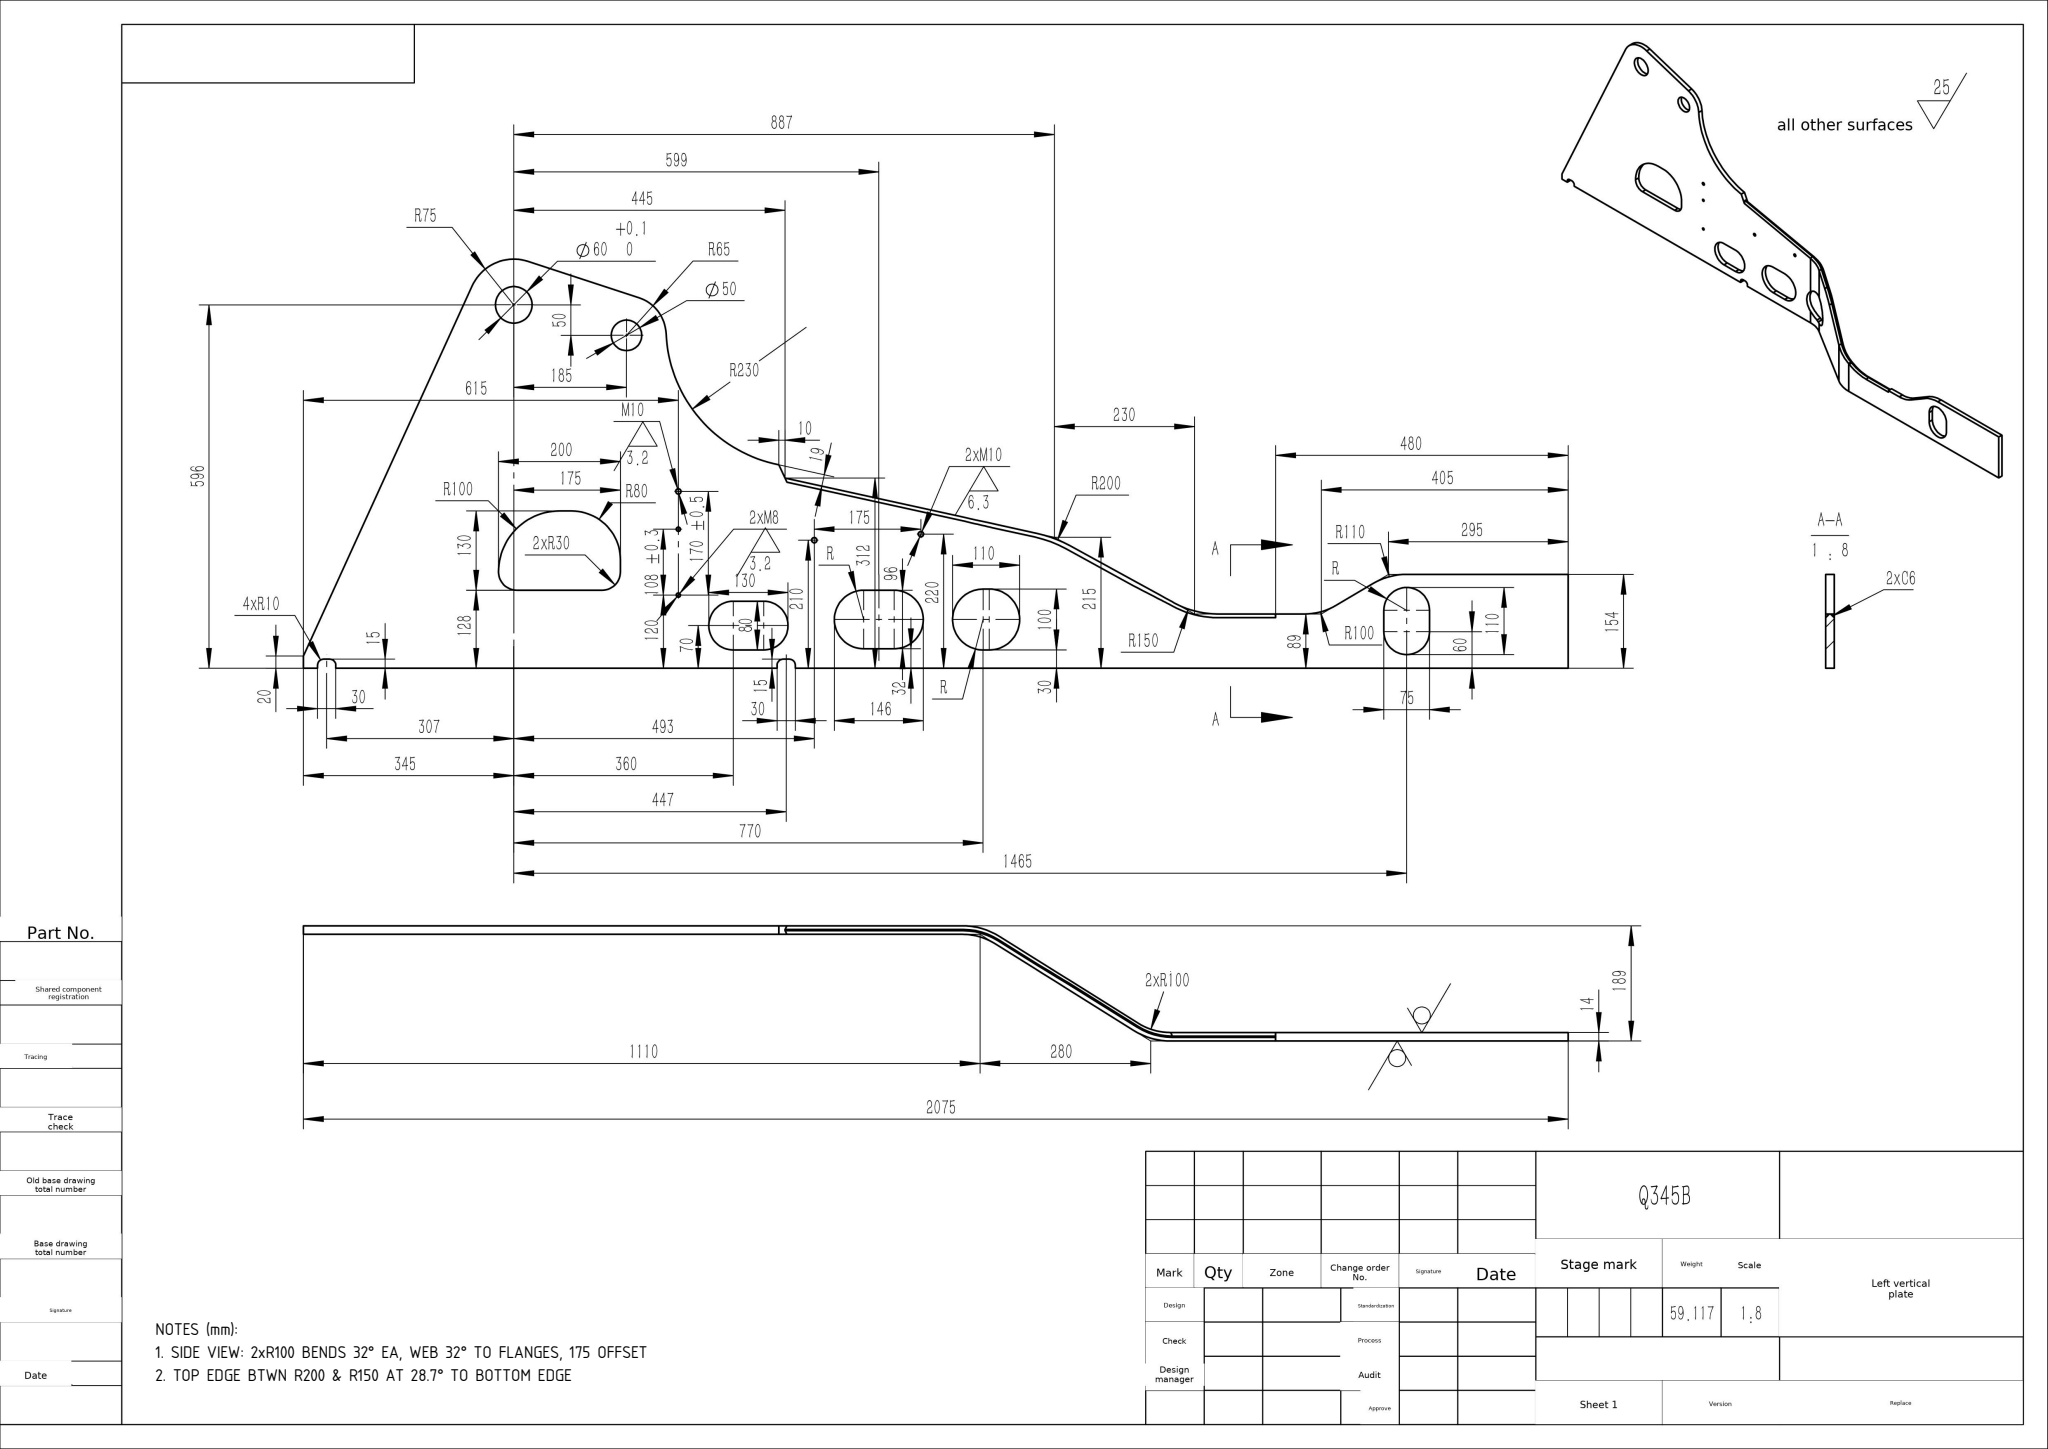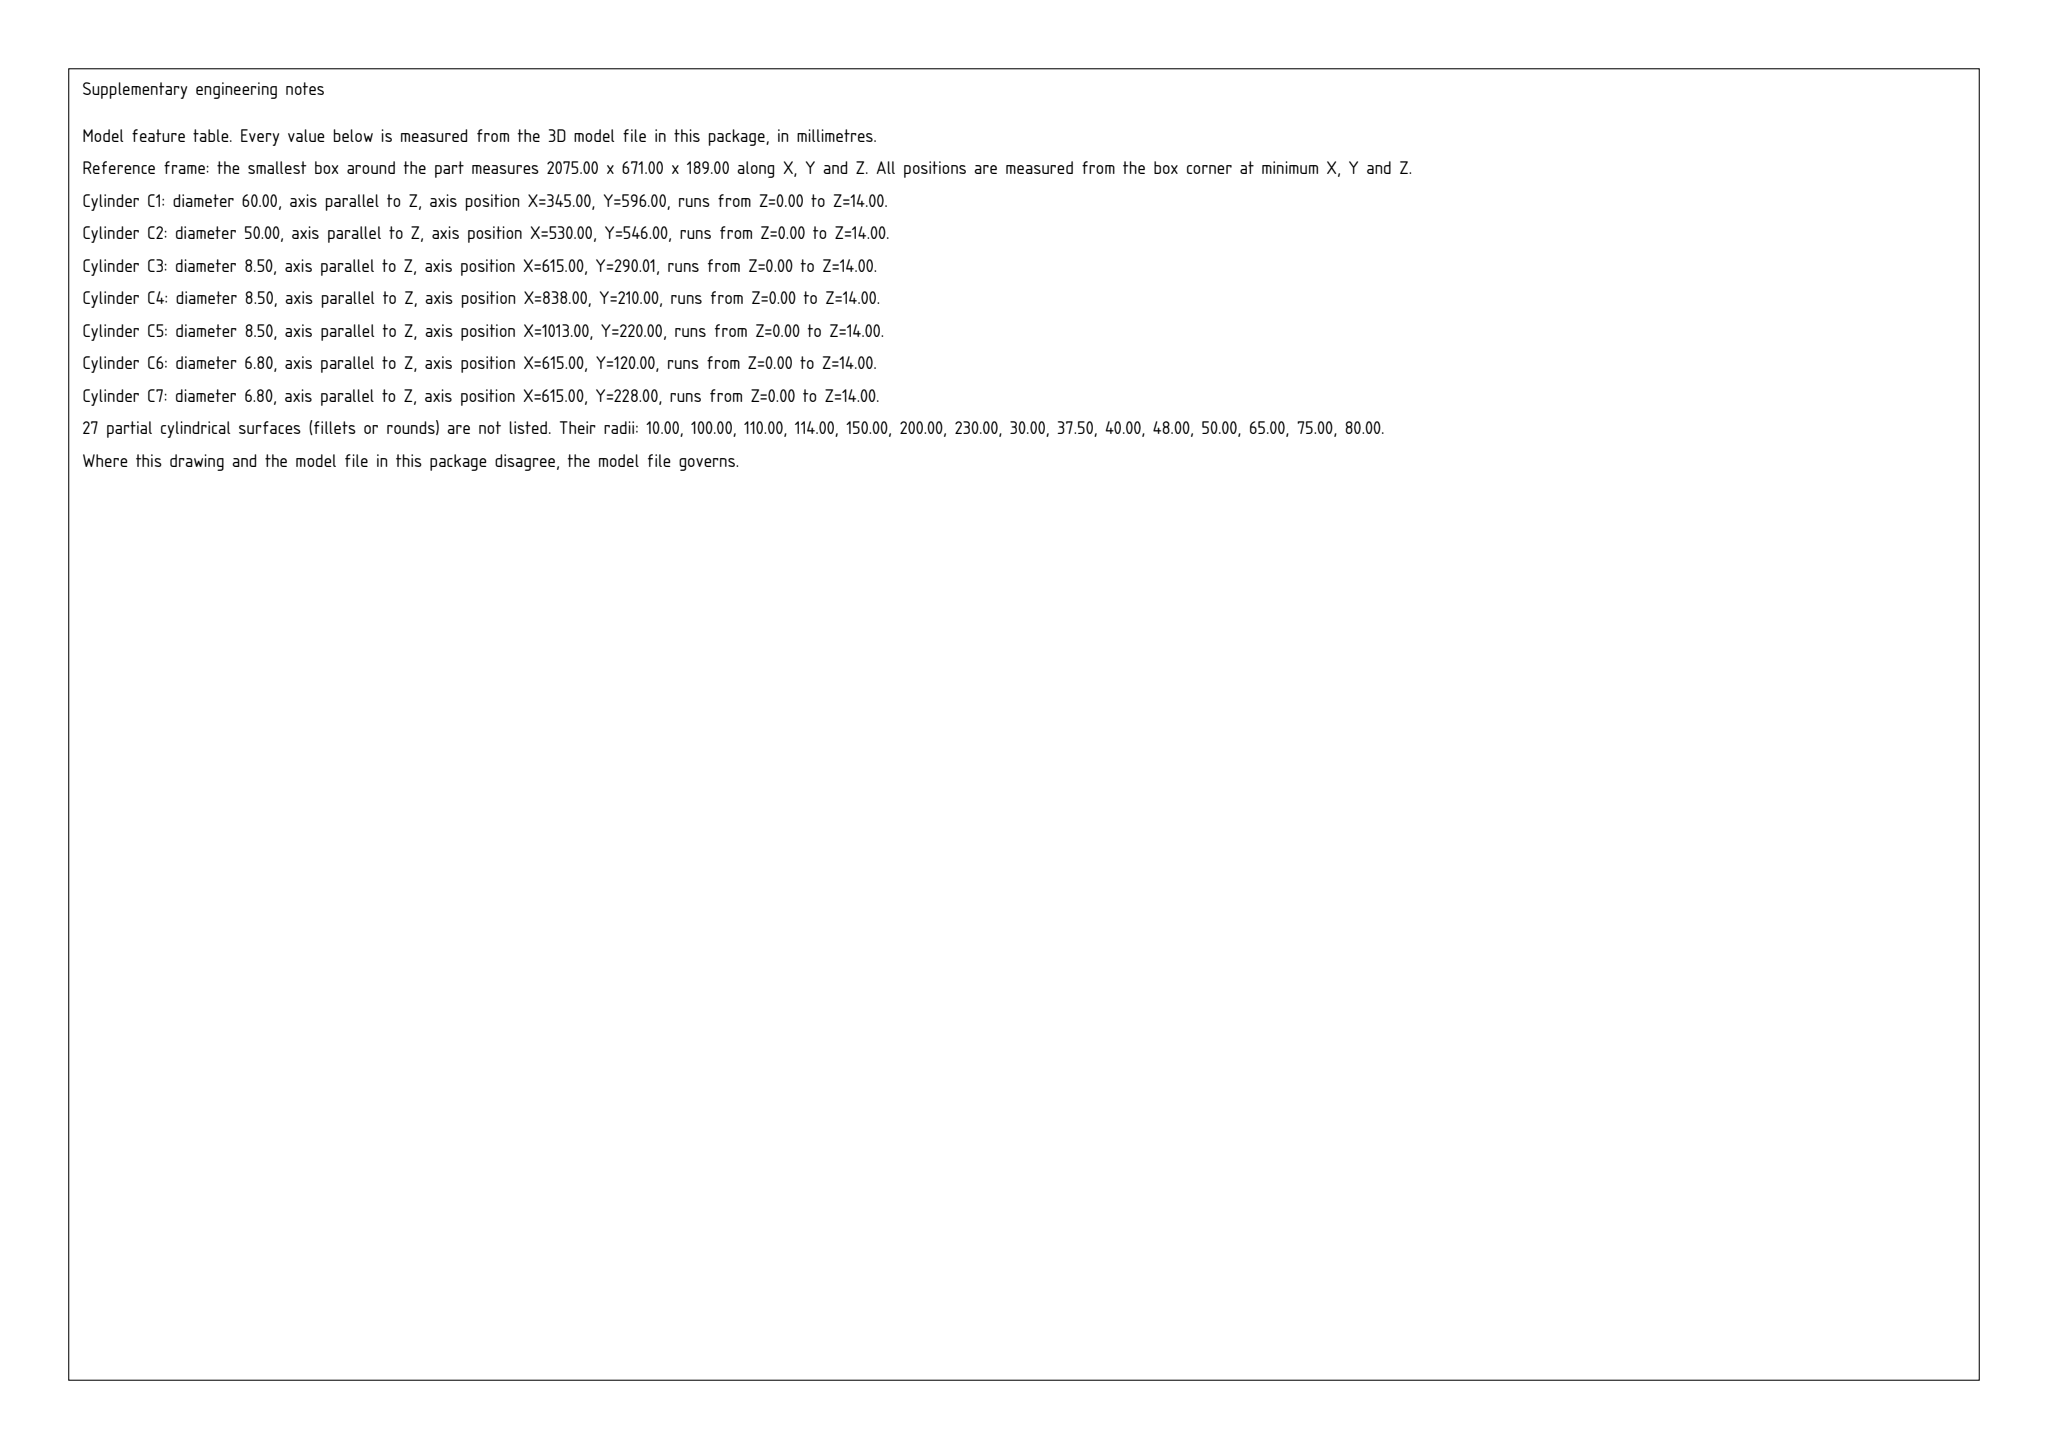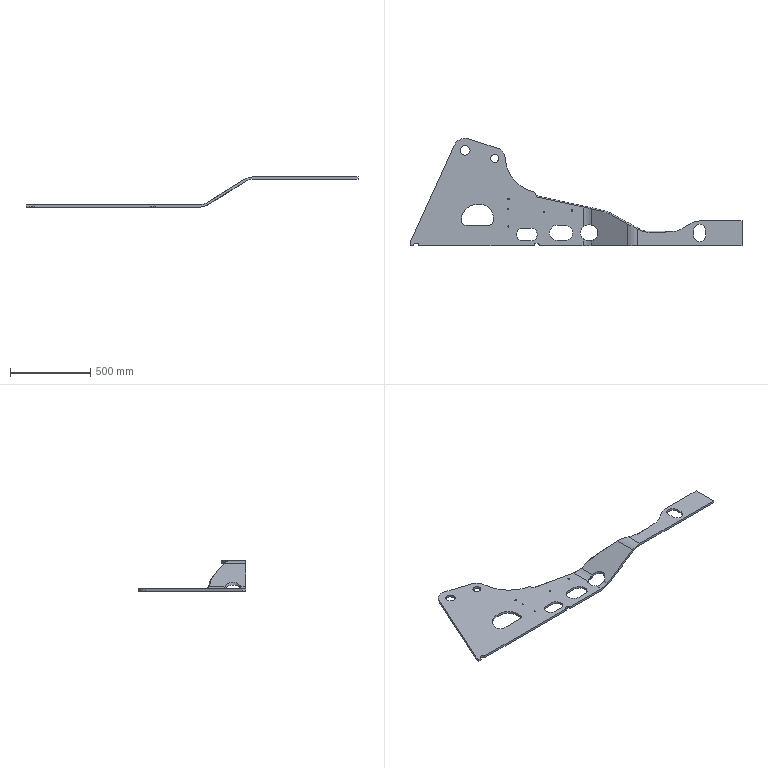Part | SolidWorks | mm | 1 solid | 103 faces | box 2075 x 671 x 189 mm | volume 7530717 mm3 | plane 49 | cylinder 46 | spline 6 | cone 2 | commonest cylinder face diameters 8.5 x6 200 x5 6.8 x4 60 x4 20 x4 80 x3 96 x3 100 x3
Drawing notes:
SIDE VIEW: 2xR100 BENDS 32° EA, WEB 32° TO FLANGES, 175 OFFSET | from the solid: Bend axes y-dia200/228 at (x1081.32,z114) and (x1422.69,z75); R100 inner/R114 outer; internal tangent gives 32.0°; face planes z=0/14 to z=175/189 (offset 175)
TOP EDGE BTWN R200 & R150 AT 28.7° TO BOTTOM EDGE | from the solid: Z-axis cyl dia400 ctr (1161.09,25.8) and dia300 ctr (1500.4,239); common tangent slope = -0.547 => 28.7° from y=0 datum edge